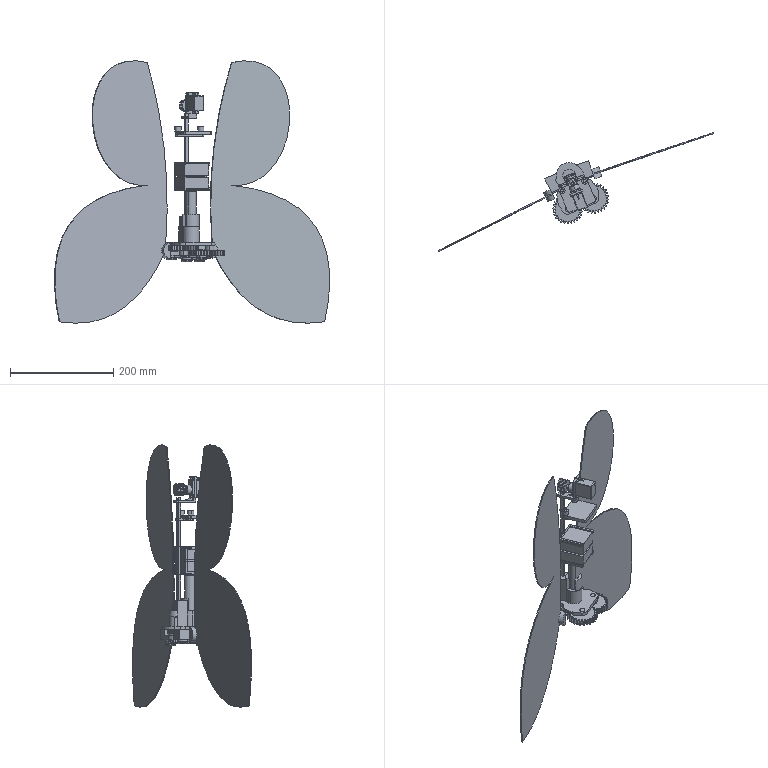Assembly | SolidWorks | mm | 32 component files | 32 solids | 771 faces | box 534.61 x 230.96 x 509.37 mm | volume 759761 mm3 | cylinder 341 | plane 260 | spline 146 | torus 16 | sphere 8 | commonest cylinder face diameters 58 x54 49 x54 10 x50 20 x40 2 x34 6 x28 28 x18 4 x14
Bill of materials:
4X4FlatKey | 1 |  | Long straight rectangular bar, a prism with a roughly square cross-section and flat ends.
Battery | 1 |  | Roughly square block with a shallow rectangular groove running around its sides at about mid-height, plus a slightly rounded edge along one side.
BatteryExoskeleton | 1 |  | Open frame made from thin bars that look like angle sections: an upper and a lower U-shaped rail joined by vertical posts at the back corners. Each rail has a small rectangular loop tab sticking out from its back member.
Collar | 2 |  | Plain cylindrical ring or sleeve with a concentric through-bore; length is less than the outer diameter.
ControlBoard | 1 |  | Thin flat plate, roughly square, with rounded corners and two round through-holes near opposite corners.
ControlSleeve | 2 |  | Cylindrical sleeve with a concentric through-bore. Its walls are thicker relative to the bore, and its length relative to diameter is greater, than in the other ring part.
CylindricalGear12x2Small | 1 |  | Straight-toothed spur-gear-like part with about 13 teeth and a central round bore with one rectangular keyway notch.
CylindricalGear27x2Large | 2 |  | Thin straight-toothed spur-gear-like disk with about 27 teeth, one central round through-hole and one second round through-hole offset from the center.
DriveShaft | 1 |  | Stepped cylindrical pin or shaft: a long main diameter that steps down to a shorter, smaller-diameter end section.
FixedMainPin42mm | 1 |  | Headed pin: a cylindrical shank with a thin, larger-diameter flange head at one end, rounded on its outer underside edge.
FixedPin14mm | 3 |  | Headed pin with a short, thick cylindrical shank and a wide head with a rounded or domed underside edge.
FixedPin24mm | 1 |  | Headed pin with a slender cylindrical shank and a flange head, rounded on the outer underside edge.
FixedPin26mm | 2 |  | Straight solid cylindrical pin with a larger-diameter domed (rounded) head at one end and a flat face at the other end.
FixedSign | 2 |  | Straight cylindrical rod with a sphere on one end and a flat, square-cut face on the other end.
Hanger | 1 |  | Flat, elongated plate with rounded corners, two cylindrical pegs rising from one face near the ends, and a side tab with a square through-opening.
MainFrame | 1 |  | Irregular flat base plate with mounting-style holes, an upright slotted tubular boss, and a long, thin, square-section rod rising beside the boss.
Sensor | 1 |  | Axisymmetric hub carrying three parallel, equally spaced circular disc flanges, with a central through-bore and a hub extension sticking out past one end disc.
SteeringController | 1 |  | Rectangular box-shaped body with rounded edges, crossed by a thin flange plate with an ear at each end; each ear has one small hole. A stepped cylindrical boss and a smaller shaft stick out from one face.
SteeringPlate | 1 |  | L-shaped bracket: an upright rectangular frame with a large rectangular window, joined by a narrower neck to a flat base plate that has a square opening.
SwingArm | 2 |  | Flat link bar of constant thickness: a ring-shaped eye with a round through-hole at each end, joined by a straight narrow web.
SwingAssistFrame(Left) | 1 |  | Stepped block with a flat tab ending in a rounded end; the tab has a large round through-hole. A semicircular channel runs along one side of the lower step.
SwingAssistFrame(Right) | 1 |  | Thin, rounded-end tab with a large round through-hole, joined to a taller rectangular block. The block has a cylindrical groove or bore along one side, and short cylindrical steps sit on the underside.
Wing | 2 |  | Very thin flat sheet with a two-lobed curved outline, with a small block and a thin pin attached at one edge.
Mates:
1. concentric | MainFrame-1 face at (28.961, 11.679, 172.846) dir (0, 0, -1) r 10 | DriveShaft-1 face at (28.961, 11.679, 240.846) dir (0, 0, -1) r 10
2. coincident | MainFrame-1 face at (-5.428, 23.48, 142.846) dir (0, 0, 1) | DriveShaft-1 face at (28.961, 11.679, 142.846) dir (0, 0, -1)
3. concentric | CylindricalGear12x2Small-1 face at (28.961, 11.679, 116.845) dir (0, 0, 1) r 5 | DriveShaft-1 face at (28.961, 11.679, 116.846) dir (0, 0, 1) r 5
4. coincident | CylindricalGear12x2Small-1 face at (28.961, 11.679, 116.846) dir (0, 0, -1) | DriveShaft-1 face at (28.961, 11.679, 116.846) dir (0, 0, -1)
5. coincident | CylindricalGear12x2Small-1 face at (25.562, 15.346, 116.846) dir (-0.4003, -0.9164, 0) | DriveShaft-1 face at (25.562, 15.346, 136.846) dir (-0.4003, -0.9164, 0)
6. coincident | CylindricalGear12x2Small-1 face at (23.961, 11.681, 116.846) dir (0.4003, 0.9164, 0) | 4X4FlatKey-1 face at (21.746, 12.648, 136.846) dir (-0.4003, -0.9164, 0)
7. coincident | DriveShaft-1 face at (25.411, 11.047, 136.846) dir (-0.9164, 0.4003, 0) | 4X4FlatKey-1 face at (25.411, 11.047, 136.846) dir (0.9164, -0.4003, 0)
8. coincident | DriveShaft-1 face at (28.961, 11.679, 116.846) dir (0, 0, -1) | 4X4FlatKey-1 face at (19.255, 25.94, 116.846) dir (0, 0, -1)
9. concentric | CylindricalGear27x2Large-2 face at (65.366, -4.894, 116.846) dir (0, 0, 1) r 5 | MainFrame-1 face at (65.366, -4.894, 136.846) dir (0, 0, 1) r 5
10. concentric | CylindricalGear27x2Large-1 face at (14.968, -25.793, 126.846) dir (0, 0, 1) r 5 | MainFrame-1 face at (14.968, -25.793, 136.846) dir (0, 0, 1) r 5
11. concentric | MainFrame-1 face at (17.47, 39.391, 136.846) dir (0, 0, 1) r 10 | SwingAssistFrame(Left)-2 face at (17.47, 39.391, 128.846) dir (0, 0, 1) r 10
12. coincident | MainFrame-1 face at (-5.428, 23.48, 136.846) dir (0, 0, -1) | SwingAssistFrame(Left)-2 face at (17.47, 39.391, 136.846) dir (0, 0, 1)
13. concentric | assembly face at (17.47, 39.391, 126.846) dir (0, 0, -1) r 10 | SwingAssistFrame(Left)-2 face at (17.47, 39.391, 128.846) dir (0, 0, 1) r 10
14. coincident | assembly face at (17.47, 39.391, 126.846) dir (0, 0, 1) | SwingAssistFrame(Left)-2 face at (17.47, 39.391, 126.846) dir (0, 0, -1)
15. concentric | MainFrame-1 face at (17.47, 39.391, 136.846) dir (0, 0, 1) r 10 | SwingAssistFrame(Right)-2 face at (17.47, 39.391, 124.846) dir (0, 0, -1) r 10
16. coincident | SwingAssistFrame(Left)-2 face at (17.47, 39.391, 124.846) dir (0, 0, -1) | SwingAssistFrame(Right)-2 face at (17.47, 39.391, 124.846) dir (0, 0, 1)
17. concentric | MainFrame-1 face at (17.47, 39.391, 136.846) dir (0, 0, 1) r 10 | FixedMainPin42mm-1 face at (17.47, 39.391, 118.846) dir (0, 0, 1) r 10
18. coincident | SwingAssistFrame(Right)-2 face at (17.47, 39.391, 114.846) dir (0, 0, -1) | FixedMainPin42mm-1 face at (17.47, 39.391, 114.846) dir (0, 0, 1)
19. coincident | SwingAssistFrame(Right)-2 face at (45.861, 49.084, 112.846) dir (0, 0, -1) | SwingArm-1 face at (21.07, -11.003, 112.846) dir (0, 0, 1)
20. concentric | CylindricalGear27x2Large-1 face at (14.968, -25.793, 126.846) dir (0, 0, 1) r 5 | FixedPin26mm-2 face at (14.968, -25.793, 116.846) dir (0, 0, 1) r 5
21. concentric | SwingArm-1 face at (45.861, 49.084, 112.846) dir (0, 0, -1) r 5 | FixedPin14mm-1 face at (45.861, 49.084, 108.846) dir (0, 0, 1) r 5
22. concentric | SwingAssistFrame(Right)-2 face at (45.861, 49.084, 126.846) dir (0, 0, -1) r 5 | FixedPin14mm-1 face at (45.861, 49.084, 108.846) dir (0, 0, 1) r 5
23. coincident | SwingArm-1 face at (21.07, -11.003, 108.846) dir (0, 0, -1) | FixedPin14mm-1 face at (45.861, 49.084, 108.846) dir (0, 0, 1)
24. concentric | CylindricalGear27x2Large-1 face at (21.07, -11.003, 126.846) dir (0, 0, 1) r 5 | FixedPin24mm-2 face at (21.07, -11.003, 108.846) dir (0, 0, 1) r 5
25. coincident | CylindricalGear27x2Large-1 face at (14.968, -25.793, 136.846) dir (0, 0, 1) | FixedPin24mm-2 face at (21.07, -11.003, 136.846) dir (0, 0, 1)
26. concentric | SwingArm-1 face at (21.07, -11.003, 112.846) dir (0, 0, -1) r 5 | FixedPin24mm-2 face at (21.07, -11.003, 108.846) dir (0, 0, 1) r 5
27. concentric | FixedPin26mm-2 face at (14.968, -25.793, 116.846) dir (0, 0, 1) r 5 | Collar-1 face at (14.968, -25.793, 126.846) dir (0, 0, -1) r 5
28. concentric | CylindricalGear27x2Large-2 face at (65.366, -4.894, 116.846) dir (0, 0, 1) r 5 | Collar-2 face at (65.366, -4.894, 136.846) dir (0, 0, -1) r 5
29. coincident | MainFrame-1 face at (-5.428, 23.48, 136.846) dir (0, 0, -1) | Collar-2 face at (65.366, -4.894, 136.846) dir (0, 0, 1)
30. concentric | CylindricalGear27x2Large-2 face at (65.366, -4.894, 116.846) dir (0, 0, 1) r 5 | FixedPin26mm-1 face at (65.366, -4.894, 116.846) dir (0, 0, 1) r 5
31. coincident | CylindricalGear27x2Large-2 face at (65.366, -4.894, 116.846) dir (0, 0, -1) | FixedPin26mm-1 face at (65.366, -4.894, 116.846) dir (0, 0, 1)
32. concentric | SwingAssistFrame(Left)-2 face at (-9.35, 25.947, 126.846) dir (0, 0, -1) r 5 | FixedPin14mm-2 face at (-9.35, 25.947, 112.846) dir (0, 0, 1) r 5
33. concentric | SwingArm-2 face at (-9.35, 25.947, 116.846) dir (0, 0, -1) r 5 | FixedPin14mm-2 face at (-9.35, 25.947, 112.846) dir (0, 0, 1) r 5
34. coincident | SwingAssistFrame(Left)-2 face at (17.47, 39.391, 116.846) dir (0, 0, -1) | SwingArm-2 face at (49.908, -0.764, 116.846) dir (0, 0, 1)
35. coincident | SwingArm-2 face at (49.908, -0.764, 112.846) dir (0, 0, -1) | FixedPin14mm-2 face at (-9.35, 25.947, 112.846) dir (0, 0, 1)
36. concentric | CylindricalGear27x2Large-2 face at (49.908, -0.764, 116.846) dir (0, 0, 1) r 5 | assembly face at (80.282, -10.682, 112.846) dir (0, 0, 1) r 5
37. concentric | SwingArm-2 face at (49.908, -0.764, 116.846) dir (0, 0, -1) r 5 | assembly face at (80.282, -10.682, 112.846) dir (0, 0, 1) r 5
38. coincident | CylindricalGear27x2Large-2 face at (65.366, -4.894, 126.846) dir (0, 0, 1) | Collar-2 face at (65.366, -4.894, 126.846) dir (0, 0, -1)
39. coincident | SwingArm-2 face at (49.908, -0.764, 112.846) dir (0, 0, -1) | assembly face at (80.282, -10.682, 112.846) dir (0, 0, 1)
40. coincident | MainFrame-1 face at (21.773, 36.845, 392.846) dir (0.9237, 0.383, 0) | BatteryExoskeleton-1 face at (24.071, 31.303, 245.846) dir (-0.9237, -0.383, 0)
41. coincident | MainFrame-1 face at (21.773, 36.845, 392.846) dir (-0.383, 0.9237, 0) | BatteryExoskeleton-1 face at (16.231, 34.547, 245.846) dir (0.383, -0.9237, 0)
42. coincident | MainFrame-1 face at (27.383, 33.759, 243.846) dir (0, 0, -1) | BatteryExoskeleton-1 face at (15.511, -26.376, 243.846) dir (0, 0, -1)
43. coincident | MainFrame-1 face at (16.231, 34.547, 392.846) dir (-0.9237, -0.383, 0) | Hanger-1 face at (16.231, 34.547, 348.846) dir (0.9237, 0.383, 0)
44. coincident | MainFrame-1 face at (21.773, 36.845, 392.846) dir (-0.383, 0.9237, 0) | Hanger-1 face at (21.773, 36.845, 348.846) dir (0.383, -0.9237, 0)
45. coincident | MainFrame-1 face at (27.766, 32.835, 352.846) dir (0, 0, 1) | Hanger-1 face at (30.222, 29.523, 352.846) dir (0, 0, 1)
46. concentric | Hanger-1 face at (3.727, 9.876, 367.846) dir (0, 0, -1) r 3 | ControlBoard-1 face at (3.727, 9.876, 358.846) dir (0, 0, -1) r 3
47. concentric | Hanger-1 face at (48.066, 28.262, 367.846) dir (0, 0, -1) r 3 | ControlBoard-1 face at (48.066, 28.262, 358.846) dir (0, 0, -1) r 3
48. coincident | Hanger-1 face at (30.222, 29.523, 352.846) dir (0, 0, 1) | ControlBoard-1 face at (66.002, -9.768, 352.846) dir (0, 0, -1)
49. concentric | Hanger-1 face at (3.727, 9.876, 367.846) dir (0, 0, -1) r 3 | ControlSleeve-1 face at (3.727, 9.876, 367.846) dir (0, 0, -1) r 3
50. coincident | ControlSleeve-1 face at (3.727, 9.876, 358.846) dir (0, 0, -1) | ControlBoard-1 face at (66.002, -9.768, 358.846) dir (0, 0, 1)
51. concentric | Hanger-1 face at (48.066, 28.262, 367.846) dir (0, 0, -1) r 3 | ControlSleeve-2 face at (48.066, 28.262, 367.846) dir (0, 0, -1) r 3
52. coincident | ControlSleeve-2 face at (48.066, 28.262, 358.846) dir (0, 0, -1) | ControlBoard-1 face at (66.002, -9.768, 358.846) dir (0, 0, 1)
53. coincident | MainFrame-1 face at (16.231, 34.547, 392.846) dir (-0.9237, -0.383, 0) | SteeringPlate-1 face at (16.231, 34.547, 383.846) dir (0.9237, 0.383, 0)
54. coincident | MainFrame-1 face at (21.773, 36.845, 392.846) dir (-0.383, 0.9237, 0) | SteeringPlate-1 face at (21.773, 36.845, 383.846) dir (0.383, -0.9237, 0)
55. coincident | MainFrame-1 face at (27.383, 33.759, 383.846) dir (0, 0, -1) | SteeringPlate-1 face at (13.617, 35.628, 383.846) dir (0, 0, -1)
56. coincident | SteeringPlate-1 face at (39.798, 6.43, 383.846) dir (0.383, -0.9237, 0) | SteeringController-1 face at (28.822, 1.878, 413.665) dir (-0.383, 0.9237, 0)
57. concentric | SteeringPlate-1 face at (30.876, 7.06, 430.346) dir (0.383, -0.9237, 0) r 1 | SteeringController-1 face at (32.409, 3.366, 430.346) dir (0.383, -0.9237, 0) r 1
58. concentric | SteeringPlate-1 face at (30.876, 7.06, 395.346) dir (0.383, -0.9237, 0) r 1 | SteeringController-1 face at (32.409, 3.366, 395.346) dir (0.383, -0.9237, 0) r 1
59. concentric | Sensor-1 face at (23.598, 24.611, 407.896) dir (0.383, -0.9237, 0) r 3 | SteeringController-1 face at (23.598, 24.611, 407.896) dir (0.383, -0.9237, 0) r 3
60. coincident | Sensor-1 face at (25.514, 19.993, 407.896) dir (0.383, -0.9237, 0) | SteeringController-1 face at (25.514, 19.993, 407.896) dir (-0.383, 0.9237, 0)
61. concentric | FixedSign-2 face at (36.622, -6.795, 395.346) dir (-0.383, 0.9237, 0) r 1 | SteeringPlate-1 face at (30.876, 7.06, 395.346) dir (0.383, -0.9237, 0) r 1
62. coincident | FixedSign-2 edge at (30.876, 7.06, 395.346) dir (-0.383, 0.9237, 0) r 1 | SteeringPlate-1 edge at (30.876, 7.06, 395.346) dir (0.383, -0.9237, 0) r 1
63. concentric | FixedSign-1 face at (36.622, -6.795, 430.346) dir (-0.383, 0.9237, 0) r 1 | SteeringPlate-1 face at (30.876, 7.06, 430.346) dir (0.383, -0.9237, 0) r 1
64. coincident | FixedSign-1 edge at (30.876, 7.06, 430.346) dir (-0.383, 0.9237, 0) r 1 | SteeringPlate-1 edge at (30.876, 7.06, 430.346) dir (0.383, -0.9237, 0) r 1
65. concentric | SwingAssistFrame(Right)-2 face at (45.975, 33.273, 126.846) dir (0.9464, 0.3231, 0) r 2 | Wing-1 face at (45.975, 33.273, 126.846) dir (0.9464, 0.3231, 0) r 2
66. parallel | SwingAssistFrame(Right)-2 face at (22.316, 25.196, 124.846) dir (0.3231, -0.9464, 0) | Wing-1 face at (67.326, 32.638, 126.846) dir (0.3231, -0.9464, 0)
67. coincident | SwingAssistFrame(Right)-2 face at (55.209, 68.126, 124.846) dir (0.9464, 0.3231, 0) | Wing-1 face at (60.864, 51.565, 141.846) dir (-0.9464, -0.3231, 0)
68. concentric | SwingAssistFrame(Left)-2 face at (1.842, 14.778, 126.846) dir (-0.894, -0.4481, 0) r 2 | Wing-2 face at (1.842, 14.778, 126.846) dir (-0.894, -0.4481, 0) r 2
69. parallel | SwingAssistFrame(Left)-2 face at (24.191, 25.981, 128.846) dir (0.4481, -0.894, 0) | Wing-2 face at (-10.436, -5.359, 126.846) dir (0.4481, -0.894, 0)
70. coincident | SwingAssistFrame(Left)-2 face at (-29.481, 32.635, 128.846) dir (-0.894, -0.4481, 0) | Wing-2 face at (-10.436, -5.359, 141.846) dir (0.894, 0.4481, 0)
71. gear | CylindricalGear27x2Large-2 edge at (65.366, -4.894, 116.846) dir (0, 0, 1) r 29 | CylindricalGear12x2Small-1 edge at (28.961, 11.679, 116.846) dir (0, 0, 1) r 14
72. gear | CylindricalGear12x2Small-1 edge at (28.961, 11.679, 116.846) dir (0, 0, 1) r 14 | CylindricalGear27x2Large-1 edge at (14.968, -25.793, 126.846) dir (0, 0, 1) r 29
73. coincident | BatteryExoskeleton-1 face at (17.358, -25.609, 295.846) dir (0.9237, 0.383, 0) | Battery-2 face at (-1.794, 20.577, 245.846) dir (-0.9237, -0.383, 0)
74. coincident | BatteryExoskeleton-1 face at (17.358, -25.609, 295.846) dir (0, 0, -1) | Battery-2 face at (-1.794, 20.577, 295.846) dir (0, 0, 1)
75. coincident | BatteryExoskeleton-1 face at (39.27, -16.523, 272.223) dir (0.383, -0.9237, 0) | Battery-2 face at (39.632, -16.373, 266.591) dir (0.383, -0.9237, 0)
76. coincident | CylindricalGear27x2Large-1 face at (14.968, -25.793, 136.846) dir (0, 0, 1) | MainFrame-1 face at (-5.428, 23.48, 136.846) dir (0, 0, -1)
77. coincident | CylindricalGear27x2Large-1 face at (14.968, -25.793, 126.846) dir (0, 0, -1) | Collar-1 face at (14.968, -25.793, 126.846) dir (0, 0, 1)
78. concentric | CylindricalGear27x2Large-2 face at (49.908, -0.764, 116.846) dir (0, 0, 1) r 5 | FixedPin14mm-3 face at (49.908, -0.764, 112.846) dir (0, 0, 1) r 5
79. concentric | SwingArm-2 face at (49.908, -0.764, 116.846) dir (0, 0, -1) r 5 | FixedPin14mm-3 face at (49.908, -0.764, 112.846) dir (0, 0, 1) r 5
80. coincident | SwingArm-2 face at (49.908, -0.764, 112.846) dir (0, 0, -1) | FixedPin14mm-3 face at (49.908, -0.764, 112.846) dir (0, 0, 1)
81. coincident | FixedPin26mm-2 face at (14.968, -25.793, 116.846) dir (0, 0, 1) | Collar-1 face at (14.968, -25.793, 116.846) dir (0, 0, -1)